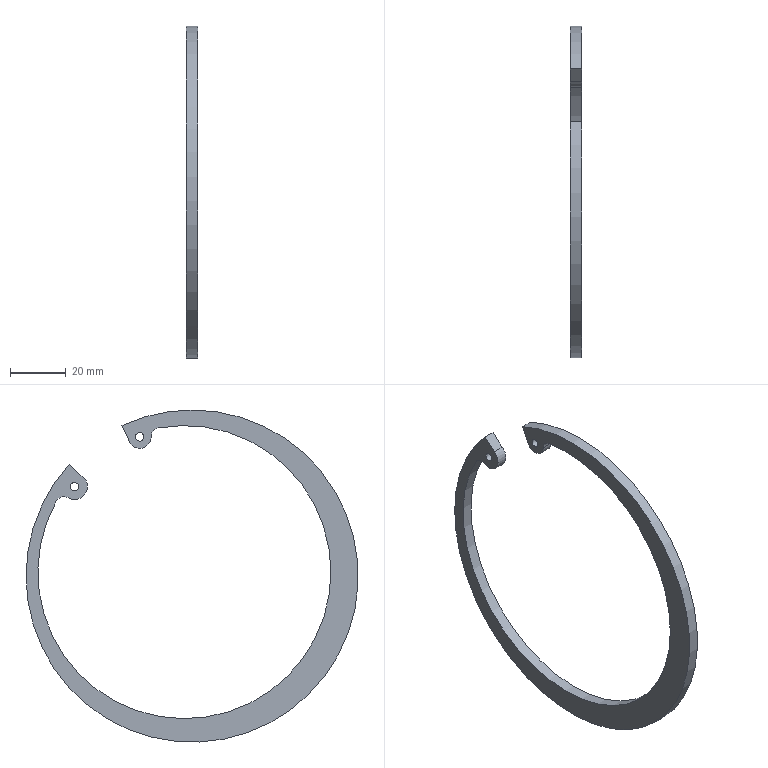Component | NX | HOLE_CLIP | 1 solid | 12 faces | box 4 x 119 x 119 mm | volume 9819 mm3 | cylinder 8 | plane 4 | commonest cylinder face diameters 6.15 x2 3 x2 8.2 x1 119 x1 9.272 x1 104.978 x1
STEP:
#1=CARTESIAN_POINT('',(0.,0.,0.));
#2=DIRECTION('',(0.,0.,1.));
#3=DIRECTION('',(1.,0.,0.));
#4=AXIS2_PLACEMENT_3D('',#1,#2,#3);
#5=CARTESIAN_POINT('',(1318.754,237.03,528.445));
#6=VERTEX_POINT('',#5);
#7=CARTESIAN_POINT('',(1314.754,237.03,528.445));
#8=VERTEX_POINT('',#7);
#9=CARTESIAN_POINT('',(1314.754,237.03,528.445));
#10=DIRECTION('',(-1.,0.,0.));
#11=VECTOR('',#10,1.);
#12=LINE('',#9,#11);
#13=CARTESIAN_POINT('',(1314.754,233.956,528.52));
#14=DIRECTION('',(1.,0.,0.));
#15=DIRECTION('',(0.,0.,-1.));
#16=AXIS2_PLACEMENT_3D('',#13,#14,#15);
#17=CYLINDRICAL_SURFACE('',#16,3.075);
#18=CARTESIAN_POINT('',(1.546,0.));
#19=DIRECTION('',(0.,-1.));
#20=VECTOR('',#19,1.);
#21=LINE('',#18,#20);
#22=(GEOMETRIC_REPRESENTATION_CONTEXT(2)PARAMETRIC_REPRESENTATION_CONTEXT()REPRESENTATION_CONTEXT('',''));
#23=DEFINITIONAL_REPRESENTATION('',(#21),#22);
#24=PCURVE('',#17,#23);
#25=CARTESIAN_POINT('',(1314.754,241.129,528.344));
#26=DIRECTION('',(1.,0.,0.));
#27=DIRECTION('',(0.,0.,-1.));
#28=AXIS2_PLACEMENT_3D('',#25,#26,#27);
#29=CYLINDRICAL_SURFACE('',#28,4.1);
#30=CARTESIAN_POINT('',(4.688,0.));
#31=DIRECTION('',(0.,-1.));
#32=VECTOR('',#31,1.);
#33=LINE('',#30,#32);
#34=(GEOMETRIC_REPRESENTATION_CONTEXT(2)PARAMETRIC_REPRESENTATION_CONTEXT()REPRESENTATION_CONTEXT('',''));
#35=DEFINITIONAL_REPRESENTATION('',(#33),#34);
#36=PCURVE('',#29,#35);
#37=SURFACE_CURVE('',#12,(#24,#36),.PCURVE_S1.);
#38=EDGE_CURVE('',#6,#8,#37,.T.);
#39=ORIENTED_EDGE('',*,*,#38,.T.);
#40=CARTESIAN_POINT('',(1314.754,234.507,531.545));
#41=VERTEX_POINT('',#40);
#42=CARTESIAN_POINT('',(1314.754,233.956,528.52));
#43=DIRECTION('',(1.,0.,0.));
#44=DIRECTION('',(0.,1.,0.));
#45=AXIS2_PLACEMENT_3D('',#42,#43,#44);
#46=CIRCLE('',#45,3.075);
#47=CARTESIAN_POINT('',(-4.712,0.));
#48=DIRECTION('',(1.,0.));
#49=VECTOR('',#48,1.);
#50=LINE('',#47,#49);
#51=(GEOMETRIC_REPRESENTATION_CONTEXT(2)PARAMETRIC_REPRESENTATION_CONTEXT()REPRESENTATION_CONTEXT('',''));
#52=DEFINITIONAL_REPRESENTATION('',(#50),#51);
#53=PCURVE('',#17,#52);
#54=CARTESIAN_POINT('',(1314.754,233.956,528.52));
#55=DIRECTION('',(-1.,0.,0.));
#56=DIRECTION('',(0.,0.,1.));
#57=AXIS2_PLACEMENT_3D('',#54,#55,#56);
#58=PLANE('',#57);
#59=CARTESIAN_POINT('',(0.,3.075));
#60=CARTESIAN_POINT('',(5.326,3.075));
#61=CARTESIAN_POINT('',(2.663,-1.538));
#62=CARTESIAN_POINT('',(0.,-6.15));
#63=CARTESIAN_POINT('',(-2.663,-1.538));
#64=CARTESIAN_POINT('',(-5.326,3.075));
#65=CARTESIAN_POINT('',(0.,3.075));
#66=(BOUNDED_CURVE()B_SPLINE_CURVE(2,(#59,#60,#61,#62,#63,#64,#65),.UNSPECIFIED.,.T.,.F.)B_SPLINE_CURVE_WITH_KNOTS((1,2,2,2,2,1),(-2.094,0.,2.094,4.189,6.283,8.378),.UNSPECIFIED.)CURVE()GEOMETRIC_REPRESENTATION_ITEM()RATIONAL_B_SPLINE_CURVE((1.,0.5,1.,0.5,1.,0.5,1.))REPRESENTATION_ITEM(''));
#67=(GEOMETRIC_REPRESENTATION_CONTEXT(2)PARAMETRIC_REPRESENTATION_CONTEXT()REPRESENTATION_CONTEXT('',''));
#68=DEFINITIONAL_REPRESENTATION('',(#66),#67);
#69=PCURVE('',#58,#68);
#70=SURFACE_CURVE('',#46,(#53,#69),.PCURVE_S1.);
#71=EDGE_CURVE('',#8,#41,#70,.T.);
#72=ORIENTED_EDGE('',*,*,#71,.T.);
#73=CARTESIAN_POINT('',(1318.754,234.507,531.545));
#74=VERTEX_POINT('',#73);
#75=CARTESIAN_POINT('',(1314.754,234.507,531.545));
#76=DIRECTION('',(-1.,0.,0.));
#77=VECTOR('',#76,1.);
#78=LINE('',#75,#77);
#79=CARTESIAN_POINT('',(2.962,0.));
#80=DIRECTION('',(0.,-1.));
#81=VECTOR('',#80,1.);
#82=LINE('',#79,#81);
#83=(GEOMETRIC_REPRESENTATION_CONTEXT(2)PARAMETRIC_REPRESENTATION_CONTEXT()REPRESENTATION_CONTEXT('',''));
#84=DEFINITIONAL_REPRESENTATION('',(#82),#83);
#85=PCURVE('',#17,#84);
#86=CARTESIAN_POINT('',(1314.754,225.111,479.904));
#87=DIRECTION('',(1.,0.,0.));
#88=DIRECTION('',(0.,0.,-1.));
#89=AXIS2_PLACEMENT_3D('',#86,#87,#88);
#90=CYLINDRICAL_SURFACE('',#89,52.489);
#91=CARTESIAN_POINT('',(2.962,0.));
#92=DIRECTION('',(0.,-1.));
#93=VECTOR('',#92,1.);
#94=LINE('',#91,#93);
#95=(GEOMETRIC_REPRESENTATION_CONTEXT(2)PARAMETRIC_REPRESENTATION_CONTEXT()REPRESENTATION_CONTEXT('',''));
#96=DEFINITIONAL_REPRESENTATION('',(#94),#95);
#97=PCURVE('',#90,#96);
#98=SURFACE_CURVE('',#78,(#85,#97),.PCURVE_S1.);
#99=EDGE_CURVE('',#74,#41,#98,.T.);
#100=ORIENTED_EDGE('',*,*,#99,.F.);
#101=CARTESIAN_POINT('',(1318.754,233.956,528.52));
#102=DIRECTION('',(1.,0.,0.));
#103=DIRECTION('',(0.,1.,0.));
#104=AXIS2_PLACEMENT_3D('',#101,#102,#103);
#105=CIRCLE('',#104,3.075);
#106=CARTESIAN_POINT('',(-4.712,4.));
#107=DIRECTION('',(1.,0.));
#108=VECTOR('',#107,1.);
#109=LINE('',#106,#108);
#110=(GEOMETRIC_REPRESENTATION_CONTEXT(2)PARAMETRIC_REPRESENTATION_CONTEXT()REPRESENTATION_CONTEXT('',''));
#111=DEFINITIONAL_REPRESENTATION('',(#109),#110);
#112=PCURVE('',#17,#111);
#113=CARTESIAN_POINT('',(1318.754,233.956,528.52));
#114=DIRECTION('',(-1.,0.,0.));
#115=DIRECTION('',(0.,0.,1.));
#116=AXIS2_PLACEMENT_3D('',#113,#114,#115);
#117=PLANE('',#116);
#118=CARTESIAN_POINT('',(0.,3.075));
#119=CARTESIAN_POINT('',(5.326,3.075));
#120=CARTESIAN_POINT('',(2.663,-1.538));
#121=CARTESIAN_POINT('',(0.,-6.15));
#122=CARTESIAN_POINT('',(-2.663,-1.538));
#123=CARTESIAN_POINT('',(-5.326,3.075));
#124=CARTESIAN_POINT('',(0.,3.075));
#125=(BOUNDED_CURVE()B_SPLINE_CURVE(2,(#118,#119,#120,#121,#122,#123,#124),.UNSPECIFIED.,.T.,.F.)B_SPLINE_CURVE_WITH_KNOTS((1,2,2,2,2,1),(-2.094,0.,2.094,4.189,6.283,8.378),.UNSPECIFIED.)CURVE()GEOMETRIC_REPRESENTATION_ITEM()RATIONAL_B_SPLINE_CURVE((1.,0.5,1.,0.5,1.,0.5,1.))REPRESENTATION_ITEM(''));
#126=(GEOMETRIC_REPRESENTATION_CONTEXT(2)PARAMETRIC_REPRESENTATION_CONTEXT()REPRESENTATION_CONTEXT('',''));
#127=DEFINITIONAL_REPRESENTATION('',(#125),#126);
#128=PCURVE('',#117,#127);
#129=SURFACE_CURVE('',#105,(#112,#128),.PCURVE_S1.);
#130=EDGE_CURVE('',#6,#74,#129,.T.);
#131=ORIENTED_EDGE('',*,*,#130,.F.);
#132=EDGE_LOOP('',(#39,#72,#100,#131));
#133=FACE_BOUND('',#132,.F.);
#134=ADVANCED_FACE('',(#133),#17,.F.);
#135=CARTESIAN_POINT('',(1318.754,244.461,525.955));
#136=VERTEX_POINT('',#135);
#137=CARTESIAN_POINT('',(1318.754,241.129,528.344));
#138=DIRECTION('',(-1.,0.,0.));
#139=DIRECTION('',(0.,1.,0.));
#140=AXIS2_PLACEMENT_3D('',#137,#138,#139);
#141=CIRCLE('',#140,4.1);
#142=CARTESIAN_POINT('',(7.854,4.));
#143=DIRECTION('',(-1.,0.));
#144=VECTOR('',#143,1.);
#145=LINE('',#142,#144);
#146=(GEOMETRIC_REPRESENTATION_CONTEXT(2)PARAMETRIC_REPRESENTATION_CONTEXT()REPRESENTATION_CONTEXT('',''));
#147=DEFINITIONAL_REPRESENTATION('',(#145),#146);
#148=PCURVE('',#29,#147);
#149=CARTESIAN_POINT('',(-0.1763,7.173));
#150=DIRECTION('',(0.,1.));
#151=AXIS2_PLACEMENT_2D('',#149,#150);
#152=CIRCLE('',#151,4.1);
#153=(GEOMETRIC_REPRESENTATION_CONTEXT(2)PARAMETRIC_REPRESENTATION_CONTEXT()REPRESENTATION_CONTEXT('',''));
#154=DEFINITIONAL_REPRESENTATION('',(#152),#153);
#155=PCURVE('',#117,#154);
#156=SURFACE_CURVE('',#141,(#148,#155),.PCURVE_S1.);
#157=EDGE_CURVE('',#136,#6,#156,.T.);
#158=ORIENTED_EDGE('',*,*,#157,.T.);
#159=ORIENTED_EDGE('',*,*,#38,.T.);
#160=CARTESIAN_POINT('',(1314.754,244.461,525.955));
#161=VERTEX_POINT('',#160);
#162=CARTESIAN_POINT('',(1314.754,241.129,528.344));
#163=DIRECTION('',(-1.,0.,0.));
#164=DIRECTION('',(0.,1.,0.));
#165=AXIS2_PLACEMENT_3D('',#162,#163,#164);
#166=CIRCLE('',#165,4.1);
#167=CARTESIAN_POINT('',(7.854,0.));
#168=DIRECTION('',(-1.,0.));
#169=VECTOR('',#168,1.);
#170=LINE('',#167,#169);
#171=(GEOMETRIC_REPRESENTATION_CONTEXT(2)PARAMETRIC_REPRESENTATION_CONTEXT()REPRESENTATION_CONTEXT('',''));
#172=DEFINITIONAL_REPRESENTATION('',(#170),#171);
#173=PCURVE('',#29,#172);
#174=CARTESIAN_POINT('',(-0.1763,7.173));
#175=DIRECTION('',(0.,1.));
#176=AXIS2_PLACEMENT_2D('',#174,#175);
#177=CIRCLE('',#176,4.1);
#178=(GEOMETRIC_REPRESENTATION_CONTEXT(2)PARAMETRIC_REPRESENTATION_CONTEXT()REPRESENTATION_CONTEXT('',''));
#179=DEFINITIONAL_REPRESENTATION('',(#177),#178);
#180=PCURVE('',#58,#179);
#181=SURFACE_CURVE('',#166,(#173,#180),.PCURVE_S1.);
#182=EDGE_CURVE('',#161,#8,#181,.T.);
#183=ORIENTED_EDGE('',*,*,#182,.F.);
#184=CARTESIAN_POINT('',(1314.754,244.461,525.955));
#185=DIRECTION('',(-1.,0.,0.));
#186=VECTOR('',#185,1.);
#187=LINE('',#184,#186);
#188=CARTESIAN_POINT('',(7.232,0.));
#189=DIRECTION('',(0.,-1.));
#190=VECTOR('',#189,1.);
#191=LINE('',#188,#190);
#192=(GEOMETRIC_REPRESENTATION_CONTEXT(2)PARAMETRIC_REPRESENTATION_CONTEXT()REPRESENTATION_CONTEXT('',''));
#193=DEFINITIONAL_REPRESENTATION('',(#191),#192);
#194=PCURVE('',#29,#193);
#195=CARTESIAN_POINT('',(1314.754,244.461,525.955));
#196=DIRECTION('',(0.,0.9065,-0.4222));
#197=DIRECTION('',(0.,0.4222,0.9065));
#198=AXIS2_PLACEMENT_3D('',#195,#196,#197);
#199=PLANE('',#198);
#200=CARTESIAN_POINT('',(0.,0.));
#201=DIRECTION('',(0.,-1.));
#202=VECTOR('',#201,1.);
#203=LINE('',#200,#202);
#204=(GEOMETRIC_REPRESENTATION_CONTEXT(2)PARAMETRIC_REPRESENTATION_CONTEXT()REPRESENTATION_CONTEXT('',''));
#205=DEFINITIONAL_REPRESENTATION('',(#203),#204);
#206=PCURVE('',#199,#205);
#207=SURFACE_CURVE('',#187,(#194,#206),.PCURVE_S1.);
#208=EDGE_CURVE('',#136,#161,#207,.T.);
#209=ORIENTED_EDGE('',*,*,#208,.F.);
#210=EDGE_LOOP('',(#158,#159,#183,#209));
#211=FACE_BOUND('',#210,.T.);
#212=ADVANCED_FACE('',(#211),#29,.T.);
#213=CARTESIAN_POINT('',(1318.754,247.47,532.414));
#214=VERTEX_POINT('',#213);
#215=CARTESIAN_POINT('',(1318.754,244.461,525.955));
#216=DIRECTION('',(0.,-0.4222,-0.9065));
#217=VECTOR('',#216,1.);
#218=LINE('',#215,#217);
#219=CARTESIAN_POINT('',(0.,4.));
#220=DIRECTION('',(-1.,0.));
#221=VECTOR('',#220,1.);
#222=LINE('',#219,#221);
#223=(GEOMETRIC_REPRESENTATION_CONTEXT(2)PARAMETRIC_REPRESENTATION_CONTEXT()REPRESENTATION_CONTEXT('',''));
#224=DEFINITIONAL_REPRESENTATION('',(#222),#223);
#225=PCURVE('',#199,#224);
#226=CARTESIAN_POINT('',(-2.565,10.505));
#227=DIRECTION('',(-0.9065,-0.4222));
#228=VECTOR('',#227,1.);
#229=LINE('',#226,#228);
#230=(GEOMETRIC_REPRESENTATION_CONTEXT(2)PARAMETRIC_REPRESENTATION_CONTEXT()REPRESENTATION_CONTEXT('',''));
#231=DEFINITIONAL_REPRESENTATION('',(#229),#230);
#232=PCURVE('',#117,#231);
#233=SURFACE_CURVE('',#218,(#225,#232),.PCURVE_S1.);
#234=EDGE_CURVE('',#214,#136,#233,.T.);
#235=ORIENTED_EDGE('',*,*,#234,.T.);
#236=ORIENTED_EDGE('',*,*,#208,.T.);
#237=CARTESIAN_POINT('',(1314.754,247.47,532.414));
#238=VERTEX_POINT('',#237);
#239=CARTESIAN_POINT('',(1314.754,244.461,525.955));
#240=DIRECTION('',(0.,-0.4222,-0.9065));
#241=VECTOR('',#240,1.);
#242=LINE('',#239,#241);
#243=CARTESIAN_POINT('',(0.,0.));
#244=DIRECTION('',(-1.,0.));
#245=VECTOR('',#244,1.);
#246=LINE('',#243,#245);
#247=(GEOMETRIC_REPRESENTATION_CONTEXT(2)PARAMETRIC_REPRESENTATION_CONTEXT()REPRESENTATION_CONTEXT('',''));
#248=DEFINITIONAL_REPRESENTATION('',(#246),#247);
#249=PCURVE('',#199,#248);
#250=CARTESIAN_POINT('',(-2.565,10.505));
#251=DIRECTION('',(-0.9065,-0.4222));
#252=VECTOR('',#251,1.);
#253=LINE('',#250,#252);
#254=(GEOMETRIC_REPRESENTATION_CONTEXT(2)PARAMETRIC_REPRESENTATION_CONTEXT()REPRESENTATION_CONTEXT('',''));
#255=DEFINITIONAL_REPRESENTATION('',(#253),#254);
#256=PCURVE('',#58,#255);
#257=SURFACE_CURVE('',#242,(#249,#256),.PCURVE_S1.);
#258=EDGE_CURVE('',#238,#161,#257,.T.);
#259=ORIENTED_EDGE('',*,*,#258,.F.);
#260=CARTESIAN_POINT('',(1314.754,247.47,532.414));
#261=DIRECTION('',(-1.,0.,0.));
#262=VECTOR('',#261,1.);
#263=LINE('',#260,#262);
#264=CARTESIAN_POINT('',(7.125,0.));
#265=DIRECTION('',(0.,-1.));
#266=VECTOR('',#265,1.);
#267=LINE('',#264,#266);
#268=(GEOMETRIC_REPRESENTATION_CONTEXT(2)PARAMETRIC_REPRESENTATION_CONTEXT()REPRESENTATION_CONTEXT('',''));
#269=DEFINITIONAL_REPRESENTATION('',(#267),#268);
#270=PCURVE('',#199,#269);
#271=CARTESIAN_POINT('',(1314.754,222.349,478.477));
#272=DIRECTION('',(1.,0.,0.));
#273=DIRECTION('',(0.,0.,-1.));
#274=AXIS2_PLACEMENT_3D('',#271,#272,#273);
#275=CYLINDRICAL_SURFACE('',#274,59.5);
#276=CARTESIAN_POINT('',(2.706,0.));
#277=DIRECTION('',(0.,-1.));
#278=VECTOR('',#277,1.);
#279=LINE('',#276,#278);
#280=(GEOMETRIC_REPRESENTATION_CONTEXT(2)PARAMETRIC_REPRESENTATION_CONTEXT()REPRESENTATION_CONTEXT('',''));
#281=DEFINITIONAL_REPRESENTATION('',(#279),#280);
#282=PCURVE('',#275,#281);
#283=SURFACE_CURVE('',#263,(#270,#282),.PCURVE_S1.);
#284=EDGE_CURVE('',#214,#238,#283,.T.);
#285=ORIENTED_EDGE('',*,*,#284,.F.);
#286=EDGE_LOOP('',(#235,#236,#259,#285));
#287=FACE_BOUND('',#286,.T.);
#288=ADVANCED_FACE('',(#287),#199,.T.);
#289=CARTESIAN_POINT('',(1318.754,266.41,518.464));
#290=VERTEX_POINT('',#289);
#291=CARTESIAN_POINT('',(1318.754,222.349,478.477));
#292=DIRECTION('',(-1.,0.,0.));
#293=DIRECTION('',(0.,1.,0.));
#294=AXIS2_PLACEMENT_3D('',#291,#292,#293);
#295=CIRCLE('',#294,59.5);
#296=CARTESIAN_POINT('',(14.137,4.));
#297=DIRECTION('',(-1.,0.));
#298=VECTOR('',#297,1.);
#299=LINE('',#296,#298);
#300=(GEOMETRIC_REPRESENTATION_CONTEXT(2)PARAMETRIC_REPRESENTATION_CONTEXT()REPRESENTATION_CONTEXT('',''));
#301=DEFINITIONAL_REPRESENTATION('',(#299),#300);
#302=PCURVE('',#275,#301);
#303=CARTESIAN_POINT('',(-50.043,-11.607));
#304=DIRECTION('',(0.,1.));
#305=AXIS2_PLACEMENT_2D('',#303,#304);
#306=CIRCLE('',#305,59.5);
#307=(GEOMETRIC_REPRESENTATION_CONTEXT(2)PARAMETRIC_REPRESENTATION_CONTEXT()REPRESENTATION_CONTEXT('',''));
#308=DEFINITIONAL_REPRESENTATION('',(#306),#307);
#309=PCURVE('',#117,#308);
#310=SURFACE_CURVE('',#295,(#302,#309),.PCURVE_S1.);
#311=EDGE_CURVE('',#290,#214,#310,.T.);
#312=ORIENTED_EDGE('',*,*,#311,.T.);
#313=ORIENTED_EDGE('',*,*,#284,.T.);
#314=CARTESIAN_POINT('',(1314.754,266.41,518.464));
#315=VERTEX_POINT('',#314);
#316=CARTESIAN_POINT('',(1314.754,222.349,478.477));
#317=DIRECTION('',(-1.,0.,0.));
#318=DIRECTION('',(0.,1.,0.));
#319=AXIS2_PLACEMENT_3D('',#316,#317,#318);
#320=CIRCLE('',#319,59.5);
#321=CARTESIAN_POINT('',(14.137,0.));
#322=DIRECTION('',(-1.,0.));
#323=VECTOR('',#322,1.);
#324=LINE('',#321,#323);
#325=(GEOMETRIC_REPRESENTATION_CONTEXT(2)PARAMETRIC_REPRESENTATION_CONTEXT()REPRESENTATION_CONTEXT('',''));
#326=DEFINITIONAL_REPRESENTATION('',(#324),#325);
#327=PCURVE('',#275,#326);
#328=CARTESIAN_POINT('',(-50.043,-11.607));
#329=DIRECTION('',(0.,1.));
#330=AXIS2_PLACEMENT_2D('',#328,#329);
#331=CIRCLE('',#330,59.5);
#332=(GEOMETRIC_REPRESENTATION_CONTEXT(2)PARAMETRIC_REPRESENTATION_CONTEXT()REPRESENTATION_CONTEXT('',''));
#333=DEFINITIONAL_REPRESENTATION('',(#331),#332);
#334=PCURVE('',#58,#333);
#335=SURFACE_CURVE('',#320,(#327,#334),.PCURVE_S1.);
#336=EDGE_CURVE('',#315,#238,#335,.T.);
#337=ORIENTED_EDGE('',*,*,#336,.F.);
#338=CARTESIAN_POINT('',(1314.754,266.41,518.464));
#339=DIRECTION('',(-1.,0.,0.));
#340=VECTOR('',#339,1.);
#341=LINE('',#338,#340);
#342=CARTESIAN_POINT('',(8.591,0.));
#343=DIRECTION('',(0.,-1.));
#344=VECTOR('',#343,1.);
#345=LINE('',#342,#344);
#346=(GEOMETRIC_REPRESENTATION_CONTEXT(2)PARAMETRIC_REPRESENTATION_CONTEXT()REPRESENTATION_CONTEXT('',''));
#347=DEFINITIONAL_REPRESENTATION('',(#345),#346);
#348=PCURVE('',#275,#347);
#349=CARTESIAN_POINT('',(1314.754,266.41,518.464));
#350=DIRECTION('',(0.,-0.672,0.7405));
#351=DIRECTION('',(0.,-0.7405,-0.672));
#352=AXIS2_PLACEMENT_3D('',#349,#350,#351);
#353=PLANE('',#352);
#354=CARTESIAN_POINT('',(0.,0.));
#355=DIRECTION('',(0.,-1.));
#356=VECTOR('',#355,1.);
#357=LINE('',#354,#356);
#358=(GEOMETRIC_REPRESENTATION_CONTEXT(2)PARAMETRIC_REPRESENTATION_CONTEXT()REPRESENTATION_CONTEXT('',''));
#359=DEFINITIONAL_REPRESENTATION('',(#357),#358);
#360=PCURVE('',#353,#359);
#361=SURFACE_CURVE('',#341,(#348,#360),.PCURVE_S1.);
#362=EDGE_CURVE('',#290,#315,#361,.T.);
#363=ORIENTED_EDGE('',*,*,#362,.F.);
#364=EDGE_LOOP('',(#312,#313,#337,#363));
#365=FACE_BOUND('',#364,.T.);
#366=ADVANCED_FACE('',(#365),#275,.T.);
#367=CARTESIAN_POINT('',(1318.754,261.776,514.258));
#368=VERTEX_POINT('',#367);
#369=CARTESIAN_POINT('',(1318.754,266.41,518.464));
#370=DIRECTION('',(-0.,0.7405,0.672));
#371=VECTOR('',#370,1.);
#372=LINE('',#369,#371);
#373=CARTESIAN_POINT('',(0.,4.));
#374=DIRECTION('',(-1.,-0.));
#375=VECTOR('',#374,1.);
#376=LINE('',#373,#375);
#377=(GEOMETRIC_REPRESENTATION_CONTEXT(2)PARAMETRIC_REPRESENTATION_CONTEXT()REPRESENTATION_CONTEXT('',''));
#378=DEFINITIONAL_REPRESENTATION('',(#376),#377);
#379=PCURVE('',#353,#378);
#380=CARTESIAN_POINT('',(-10.056,32.453));
#381=DIRECTION('',(0.672,0.7405));
#382=VECTOR('',#381,1.);
#383=LINE('',#380,#382);
#384=(GEOMETRIC_REPRESENTATION_CONTEXT(2)PARAMETRIC_REPRESENTATION_CONTEXT()REPRESENTATION_CONTEXT('',''));
#385=DEFINITIONAL_REPRESENTATION('',(#383),#384);
#386=PCURVE('',#117,#385);
#387=SURFACE_CURVE('',#372,(#379,#386),.PCURVE_S1.);
#388=EDGE_CURVE('',#368,#290,#387,.T.);
#389=ORIENTED_EDGE('',*,*,#388,.T.);
#390=ORIENTED_EDGE('',*,*,#362,.T.);
#391=CARTESIAN_POINT('',(1314.754,261.776,514.258));
#392=VERTEX_POINT('',#391);
#393=CARTESIAN_POINT('',(1314.754,266.41,518.464));
#394=DIRECTION('',(-0.,0.7405,0.672));
#395=VECTOR('',#394,1.);
#396=LINE('',#393,#395);
#397=CARTESIAN_POINT('',(0.,0.));
#398=DIRECTION('',(-1.,-0.));
#399=VECTOR('',#398,1.);
#400=LINE('',#397,#399);
#401=(GEOMETRIC_REPRESENTATION_CONTEXT(2)PARAMETRIC_REPRESENTATION_CONTEXT()REPRESENTATION_CONTEXT('',''));
#402=DEFINITIONAL_REPRESENTATION('',(#400),#401);
#403=PCURVE('',#353,#402);
#404=CARTESIAN_POINT('',(-10.056,32.453));
#405=DIRECTION('',(0.672,0.7405));
#406=VECTOR('',#405,1.);
#407=LINE('',#404,#406);
#408=(GEOMETRIC_REPRESENTATION_CONTEXT(2)PARAMETRIC_REPRESENTATION_CONTEXT()REPRESENTATION_CONTEXT('',''));
#409=DEFINITIONAL_REPRESENTATION('',(#407),#408);
#410=PCURVE('',#58,#409);
#411=SURFACE_CURVE('',#396,(#403,#410),.PCURVE_S1.);
#412=EDGE_CURVE('',#392,#315,#411,.T.);
#413=ORIENTED_EDGE('',*,*,#412,.F.);
#414=CARTESIAN_POINT('',(1314.754,261.776,514.258));
#415=DIRECTION('',(-1.,0.,0.));
#416=VECTOR('',#415,1.);
#417=LINE('',#414,#416);
#418=CARTESIAN_POINT('',(6.258,0.));
#419=DIRECTION('',(0.,-1.));
#420=VECTOR('',#419,1.);
#421=LINE('',#418,#420);
#422=(GEOMETRIC_REPRESENTATION_CONTEXT(2)PARAMETRIC_REPRESENTATION_CONTEXT()REPRESENTATION_CONTEXT('',''));
#423=DEFINITIONAL_REPRESENTATION('',(#421),#422);
#424=PCURVE('',#353,#423);
#425=CARTESIAN_POINT('',(1314.754,264.515,510.518));
#426=DIRECTION('',(1.,0.,0.));
#427=DIRECTION('',(0.,0.,-1.));
#428=AXIS2_PLACEMENT_3D('',#425,#426,#427);
#429=CYLINDRICAL_SURFACE('',#428,4.636);
#430=CARTESIAN_POINT('',(3.774,0.));
#431=DIRECTION('',(0.,-1.));
#432=VECTOR('',#431,1.);
#433=LINE('',#430,#432);
#434=(GEOMETRIC_REPRESENTATION_CONTEXT(2)PARAMETRIC_REPRESENTATION_CONTEXT()REPRESENTATION_CONTEXT('',''));
#435=DEFINITIONAL_REPRESENTATION('',(#433),#434);
#436=PCURVE('',#429,#435);
#437=SURFACE_CURVE('',#417,(#424,#436),.PCURVE_S1.);
#438=EDGE_CURVE('',#368,#392,#437,.T.);
#439=ORIENTED_EDGE('',*,*,#438,.F.);
#440=EDGE_LOOP('',(#389,#390,#413,#439));
#441=FACE_BOUND('',#440,.T.);
#442=ADVANCED_FACE('',(#441),#353,.T.);
#443=CARTESIAN_POINT('',(1318.754,267.254,506.778));
#444=VERTEX_POINT('',#443);
#445=CARTESIAN_POINT('',(1318.754,264.515,510.518));
#446=DIRECTION('',(-1.,0.,0.));
#447=DIRECTION('',(0.,1.,0.));
#448=AXIS2_PLACEMENT_3D('',#445,#446,#447);
#449=CIRCLE('',#448,4.636);
#450=CARTESIAN_POINT('',(7.854,4.));
#451=DIRECTION('',(-1.,0.));
#452=VECTOR('',#451,1.);
#453=LINE('',#450,#452);
#454=(GEOMETRIC_REPRESENTATION_CONTEXT(2)PARAMETRIC_REPRESENTATION_CONTEXT()REPRESENTATION_CONTEXT('',''));
#455=DEFINITIONAL_REPRESENTATION('',(#453),#454);
#456=PCURVE('',#429,#455);
#457=CARTESIAN_POINT('',(-18.002,30.559));
#458=DIRECTION('',(0.,1.));
#459=AXIS2_PLACEMENT_2D('',#457,#458);
#460=CIRCLE('',#459,4.636);
#461=(GEOMETRIC_REPRESENTATION_CONTEXT(2)PARAMETRIC_REPRESENTATION_CONTEXT()REPRESENTATION_CONTEXT('',''));
#462=DEFINITIONAL_REPRESENTATION('',(#460),#461);
#463=PCURVE('',#117,#462);
#464=SURFACE_CURVE('',#449,(#456,#463),.PCURVE_S1.);
#465=EDGE_CURVE('',#444,#368,#464,.T.);
#466=ORIENTED_EDGE('',*,*,#465,.T.);
#467=ORIENTED_EDGE('',*,*,#438,.T.);
#468=CARTESIAN_POINT('',(1314.754,267.254,506.778));
#469=VERTEX_POINT('',#468);
#470=CARTESIAN_POINT('',(1314.754,264.515,510.518));
#471=DIRECTION('',(-1.,0.,0.));
#472=DIRECTION('',(0.,1.,0.));
#473=AXIS2_PLACEMENT_3D('',#470,#471,#472);
#474=CIRCLE('',#473,4.636);
#475=CARTESIAN_POINT('',(7.854,0.));
#476=DIRECTION('',(-1.,0.));
#477=VECTOR('',#476,1.);
#478=LINE('',#475,#477);
#479=(GEOMETRIC_REPRESENTATION_CONTEXT(2)PARAMETRIC_REPRESENTATION_CONTEXT()REPRESENTATION_CONTEXT('',''));
#480=DEFINITIONAL_REPRESENTATION('',(#478),#479);
#481=PCURVE('',#429,#480);
#482=CARTESIAN_POINT('',(-18.002,30.559));
#483=DIRECTION('',(0.,1.));
#484=AXIS2_PLACEMENT_2D('',#482,#483);
#485=CIRCLE('',#484,4.636);
#486=(GEOMETRIC_REPRESENTATION_CONTEXT(2)PARAMETRIC_REPRESENTATION_CONTEXT()REPRESENTATION_CONTEXT('',''));
#487=DEFINITIONAL_REPRESENTATION('',(#485),#486);
#488=PCURVE('',#58,#487);
#489=SURFACE_CURVE('',#474,(#481,#488),.PCURVE_S1.);
#490=EDGE_CURVE('',#469,#392,#489,.T.);
#491=ORIENTED_EDGE('',*,*,#490,.F.);
#492=CARTESIAN_POINT('',(1314.754,267.254,506.778));
#493=DIRECTION('',(-1.,0.,0.));
#494=VECTOR('',#493,1.);
#495=LINE('',#492,#494);
#496=CARTESIAN_POINT('',(6.915,0.));
#497=DIRECTION('',(0.,-1.));
#498=VECTOR('',#497,1.);
#499=LINE('',#496,#498);
#500=(GEOMETRIC_REPRESENTATION_CONTEXT(2)PARAMETRIC_REPRESENTATION_CONTEXT()REPRESENTATION_CONTEXT('',''));
#501=DEFINITIONAL_REPRESENTATION('',(#499),#500);
#502=PCURVE('',#429,#501);
#503=CARTESIAN_POINT('',(1314.754,268.313,503.891));
#504=DIRECTION('',(1.,0.,0.));
#505=DIRECTION('',(0.,0.,-1.));
#506=AXIS2_PLACEMENT_3D('',#503,#504,#505);
#507=CYLINDRICAL_SURFACE('',#506,3.075);
#508=CARTESIAN_POINT('',(3.493,0.));
#509=DIRECTION('',(0.,-1.));
#510=VECTOR('',#509,1.);
#511=LINE('',#508,#510);
#512=(GEOMETRIC_REPRESENTATION_CONTEXT(2)PARAMETRIC_REPRESENTATION_CONTEXT()REPRESENTATION_CONTEXT('',''));
#513=DEFINITIONAL_REPRESENTATION('',(#511),#512);
#514=PCURVE('',#507,#513);
#515=SURFACE_CURVE('',#495,(#502,#514),.PCURVE_S1.);
#516=EDGE_CURVE('',#444,#469,#515,.T.);
#517=ORIENTED_EDGE('',*,*,#516,.F.);
#518=EDGE_LOOP('',(#466,#467,#491,#517));
#519=FACE_BOUND('',#518,.T.);
#520=ADVANCED_FACE('',(#519),#429,.T.);
#521=CARTESIAN_POINT('',(1318.754,271.001,505.383));
#522=VERTEX_POINT('',#521);
#523=CARTESIAN_POINT('',(1314.754,271.001,505.383));
#524=VERTEX_POINT('',#523);
#525=CARTESIAN_POINT('',(1314.754,271.001,505.383));
#526=DIRECTION('',(-1.,0.,0.));
#527=VECTOR('',#526,1.);
#528=LINE('',#525,#527);
#529=CARTESIAN_POINT('',(2.078,0.));
#530=DIRECTION('',(0.,-1.));
#531=VECTOR('',#530,1.);
#532=LINE('',#529,#531);
#533=(GEOMETRIC_REPRESENTATION_CONTEXT(2)PARAMETRIC_REPRESENTATION_CONTEXT()REPRESENTATION_CONTEXT('',''));
#534=DEFINITIONAL_REPRESENTATION('',(#532),#533);
#535=PCURVE('',#507,#534);
#536=CARTESIAN_POINT('',(8.361,0.));
#537=DIRECTION('',(0.,-1.));
#538=VECTOR('',#537,1.);
#539=LINE('',#536,#538);
#540=(GEOMETRIC_REPRESENTATION_CONTEXT(2)PARAMETRIC_REPRESENTATION_CONTEXT()REPRESENTATION_CONTEXT('',''));
#541=DEFINITIONAL_REPRESENTATION('',(#539),#540);
#542=PCURVE('',#90,#541);
#543=SURFACE_CURVE('',#528,(#535,#542),.PCURVE_S1.);
#544=EDGE_CURVE('',#522,#524,#543,.T.);
#545=ORIENTED_EDGE('',*,*,#544,.T.);
#546=CARTESIAN_POINT('',(1314.754,268.313,503.891));
#547=DIRECTION('',(1.,0.,0.));
#548=DIRECTION('',(0.,1.,0.));
#549=AXIS2_PLACEMENT_3D('',#546,#547,#548);
#550=CIRCLE('',#549,3.075);
#551=CARTESIAN_POINT('',(1.571,0.));
#552=DIRECTION('',(1.,0.));
#553=VECTOR('',#552,1.);
#554=LINE('',#551,#553);
#555=(GEOMETRIC_REPRESENTATION_CONTEXT(2)PARAMETRIC_REPRESENTATION_CONTEXT()REPRESENTATION_CONTEXT('',''));
#556=DEFINITIONAL_REPRESENTATION('',(#554),#555);
#557=PCURVE('',#507,#556);
#558=CARTESIAN_POINT('',(-24.63,37.432));
#559=CARTESIAN_POINT('',(-19.303,37.432));
#560=CARTESIAN_POINT('',(-21.966,32.819));
#561=CARTESIAN_POINT('',(-24.63,28.207));
#562=CARTESIAN_POINT('',(-27.293,32.819));
#563=CARTESIAN_POINT('',(-29.956,37.432));
#564=CARTESIAN_POINT('',(-24.63,37.432));
#565=(BOUNDED_CURVE()B_SPLINE_CURVE(2,(#558,#559,#560,#561,#562,#563,#564),.UNSPECIFIED.,.T.,.F.)B_SPLINE_CURVE_WITH_KNOTS((1,2,2,2,2,1),(-2.094,0.,2.094,4.189,6.283,8.378),.UNSPECIFIED.)CURVE()GEOMETRIC_REPRESENTATION_ITEM()RATIONAL_B_SPLINE_CURVE((1.,0.5,1.,0.5,1.,0.5,1.))REPRESENTATION_ITEM(''));
#566=(GEOMETRIC_REPRESENTATION_CONTEXT(2)PARAMETRIC_REPRESENTATION_CONTEXT()REPRESENTATION_CONTEXT('',''));
#567=DEFINITIONAL_REPRESENTATION('',(#565),#566);
#568=PCURVE('',#58,#567);
#569=SURFACE_CURVE('',#550,(#557,#568),.PCURVE_S1.);
#570=EDGE_CURVE('',#524,#469,#569,.T.);
#571=ORIENTED_EDGE('',*,*,#570,.T.);
#572=ORIENTED_EDGE('',*,*,#516,.F.);
#573=CARTESIAN_POINT('',(1318.754,268.313,503.891));
#574=DIRECTION('',(1.,0.,0.));
#575=DIRECTION('',(0.,1.,0.));
#576=AXIS2_PLACEMENT_3D('',#573,#574,#575);
#577=CIRCLE('',#576,3.075);
#578=CARTESIAN_POINT('',(1.571,4.));
#579=DIRECTION('',(1.,0.));
#580=VECTOR('',#579,1.);
#581=LINE('',#578,#580);
#582=(GEOMETRIC_REPRESENTATION_CONTEXT(2)PARAMETRIC_REPRESENTATION_CONTEXT()REPRESENTATION_CONTEXT('',''));
#583=DEFINITIONAL_REPRESENTATION('',(#581),#582);
#584=PCURVE('',#507,#583);
#585=CARTESIAN_POINT('',(-24.63,37.432));
#586=CARTESIAN_POINT('',(-19.303,37.432));
#587=CARTESIAN_POINT('',(-21.966,32.819));
#588=CARTESIAN_POINT('',(-24.63,28.207));
#589=CARTESIAN_POINT('',(-27.293,32.819));
#590=CARTESIAN_POINT('',(-29.956,37.432));
#591=CARTESIAN_POINT('',(-24.63,37.432));
#592=(BOUNDED_CURVE()B_SPLINE_CURVE(2,(#585,#586,#587,#588,#589,#590,#591),.UNSPECIFIED.,.T.,.F.)B_SPLINE_CURVE_WITH_KNOTS((1,2,2,2,2,1),(-2.094,0.,2.094,4.189,6.283,8.378),.UNSPECIFIED.)CURVE()GEOMETRIC_REPRESENTATION_ITEM()RATIONAL_B_SPLINE_CURVE((1.,0.5,1.,0.5,1.,0.5,1.))REPRESENTATION_ITEM(''));
#593=(GEOMETRIC_REPRESENTATION_CONTEXT(2)PARAMETRIC_REPRESENTATION_CONTEXT()REPRESENTATION_CONTEXT('',''));
#594=DEFINITIONAL_REPRESENTATION('',(#592),#593);
#595=PCURVE('',#117,#594);
#596=SURFACE_CURVE('',#577,(#584,#595),.PCURVE_S1.);
#597=EDGE_CURVE('',#522,#444,#596,.T.);
#598=ORIENTED_EDGE('',*,*,#597,.F.);
#599=EDGE_LOOP('',(#545,#571,#572,#598));
#600=FACE_BOUND('',#599,.F.);
#601=ADVANCED_FACE('',(#600),#507,.F.);
#602=CARTESIAN_POINT('',(1314.754,242.629,528.344));
#603=VERTEX_POINT('',#602);
#604=CARTESIAN_POINT('',(1314.754,241.129,528.344));
#605=DIRECTION('',(-1.,0.,0.));
#606=DIRECTION('',(0.,1.,0.));
#607=AXIS2_PLACEMENT_3D('',#604,#605,#606);
#608=CIRCLE('',#607,1.5);
#609=CARTESIAN_POINT('',(1314.754,241.129,528.344));
#610=DIRECTION('',(1.,0.,0.));
#611=DIRECTION('',(0.,0.,-1.));
#612=AXIS2_PLACEMENT_3D('',#609,#610,#611);
#613=CYLINDRICAL_SURFACE('',#612,1.5);
#614=CARTESIAN_POINT('',(7.854,0.));
#615=DIRECTION('',(-1.,0.));
#616=VECTOR('',#615,1.);
#617=LINE('',#614,#616);
#618=(GEOMETRIC_REPRESENTATION_CONTEXT(2)PARAMETRIC_REPRESENTATION_CONTEXT()REPRESENTATION_CONTEXT('',''));
#619=DEFINITIONAL_REPRESENTATION('',(#617),#618);
#620=PCURVE('',#613,#619);
#621=CARTESIAN_POINT('',(-0.1763,7.173));
#622=DIRECTION('',(0.,1.));
#623=AXIS2_PLACEMENT_2D('',#621,#622);
#624=CIRCLE('',#623,1.5);
#625=(GEOMETRIC_REPRESENTATION_CONTEXT(2)PARAMETRIC_REPRESENTATION_CONTEXT()REPRESENTATION_CONTEXT('',''));
#626=DEFINITIONAL_REPRESENTATION('',(#624),#625);
#627=PCURVE('',#58,#626);
#628=SURFACE_CURVE('',#608,(#620,#627),.PCURVE_S1.);
#629=EDGE_CURVE('',#603,#603,#628,.T.);
#630=ORIENTED_EDGE('',*,*,#629,.F.);
#631=CARTESIAN_POINT('',(1318.754,242.629,528.344));
#632=VERTEX_POINT('',#631);
#633=CARTESIAN_POINT('',(1314.754,242.629,528.344));
#634=CARTESIAN_POINT('',(1318.754,242.629,528.344));
#635=B_SPLINE_CURVE_WITH_KNOTS('',1,(#633,#634),.UNSPECIFIED.,.F.,.F.,(2,2),(0.,4.),.PIECEWISE_BEZIER_KNOTS.);
#636=CARTESIAN_POINT('',(7.854,0.));
#637=DIRECTION('',(0.,1.));
#638=VECTOR('',#637,1.);
#639=LINE('',#636,#638);
#640=(GEOMETRIC_REPRESENTATION_CONTEXT(2)PARAMETRIC_REPRESENTATION_CONTEXT()REPRESENTATION_CONTEXT('',''));
#641=DEFINITIONAL_REPRESENTATION('',(#639),#640);
#642=PCURVE('',#613,#641);
#643=CARTESIAN_POINT('',(1.571,0.));
#644=DIRECTION('',(0.,1.));
#645=VECTOR('',#644,1.);
#646=LINE('',#643,#645);
#647=(GEOMETRIC_REPRESENTATION_CONTEXT(2)PARAMETRIC_REPRESENTATION_CONTEXT()REPRESENTATION_CONTEXT('',''));
#648=DEFINITIONAL_REPRESENTATION('',(#646),#647);
#649=PCURVE('',#613,#648);
#650=SEAM_CURVE('',#635,(#642,#649),.PCURVE_S1.);
#651=EDGE_CURVE('',#603,#632,#650,.T.);
#652=ORIENTED_EDGE('',*,*,#651,.T.);
#653=CARTESIAN_POINT('',(1318.754,241.129,528.344));
#654=DIRECTION('',(-1.,0.,0.));
#655=DIRECTION('',(0.,1.,0.));
#656=AXIS2_PLACEMENT_3D('',#653,#654,#655);
#657=CIRCLE('',#656,1.5);
#658=CARTESIAN_POINT('',(7.854,4.));
#659=DIRECTION('',(-1.,0.));
#660=VECTOR('',#659,1.);
#661=LINE('',#658,#660);
#662=(GEOMETRIC_REPRESENTATION_CONTEXT(2)PARAMETRIC_REPRESENTATION_CONTEXT()REPRESENTATION_CONTEXT('',''));
#663=DEFINITIONAL_REPRESENTATION('',(#661),#662);
#664=PCURVE('',#613,#663);
#665=CARTESIAN_POINT('',(-0.1763,7.173));
#666=DIRECTION('',(0.,1.));
#667=AXIS2_PLACEMENT_2D('',#665,#666);
#668=CIRCLE('',#667,1.5);
#669=(GEOMETRIC_REPRESENTATION_CONTEXT(2)PARAMETRIC_REPRESENTATION_CONTEXT()REPRESENTATION_CONTEXT('',''));
#670=DEFINITIONAL_REPRESENTATION('',(#668),#669);
#671=PCURVE('',#117,#670);
#672=SURFACE_CURVE('',#657,(#664,#671),.PCURVE_S1.);
#673=EDGE_CURVE('',#632,#632,#672,.T.);
#674=ORIENTED_EDGE('',*,*,#673,.T.);
#675=ORIENTED_EDGE('',*,*,#651,.F.);
#676=EDGE_LOOP('',(#630,#652,#674,#675));
#677=FACE_BOUND('',#676,.F.);
#678=ADVANCED_FACE('',(#677),#613,.F.);
#679=ORIENTED_EDGE('',*,*,#99,.T.);
#680=CARTESIAN_POINT('',(1314.754,225.111,479.904));
#681=DIRECTION('',(1.,0.,0.));
#682=DIRECTION('',(0.,1.,0.));
#683=AXIS2_PLACEMENT_3D('',#680,#681,#682);
#684=CIRCLE('',#683,52.489);
#685=CARTESIAN_POINT('',(1.571,0.));
#686=DIRECTION('',(1.,0.));
#687=VECTOR('',#686,1.);
#688=LINE('',#685,#687);
#689=(GEOMETRIC_REPRESENTATION_CONTEXT(2)PARAMETRIC_REPRESENTATION_CONTEXT()REPRESENTATION_CONTEXT('',''));
#690=DEFINITIONAL_REPRESENTATION('',(#688),#689);
#691=PCURVE('',#90,#690);
#692=CARTESIAN_POINT('',(-48.616,43.644));
#693=CARTESIAN_POINT('',(42.298,43.644));
#694=CARTESIAN_POINT('',(-3.159,-35.09));
#695=CARTESIAN_POINT('',(-48.616,-113.823));
#696=CARTESIAN_POINT('',(-94.072,-35.09));
#697=CARTESIAN_POINT('',(-139.529,43.644));
#698=CARTESIAN_POINT('',(-48.616,43.644));
#699=(BOUNDED_CURVE()B_SPLINE_CURVE(2,(#692,#693,#694,#695,#696,#697,#698),.UNSPECIFIED.,.T.,.F.)B_SPLINE_CURVE_WITH_KNOTS((1,2,2,2,2,1),(-2.094,0.,2.094,4.189,6.283,8.378),.UNSPECIFIED.)CURVE()GEOMETRIC_REPRESENTATION_ITEM()RATIONAL_B_SPLINE_CURVE((1.,0.5,1.,0.5,1.,0.5,1.))REPRESENTATION_ITEM(''));
#700=(GEOMETRIC_REPRESENTATION_CONTEXT(2)PARAMETRIC_REPRESENTATION_CONTEXT()REPRESENTATION_CONTEXT('',''));
#701=DEFINITIONAL_REPRESENTATION('',(#699),#700);
#702=PCURVE('',#58,#701);
#703=SURFACE_CURVE('',#684,(#691,#702),.PCURVE_S1.);
#704=EDGE_CURVE('',#41,#524,#703,.T.);
#705=ORIENTED_EDGE('',*,*,#704,.T.);
#706=ORIENTED_EDGE('',*,*,#544,.F.);
#707=CARTESIAN_POINT('',(1318.754,225.111,479.904));
#708=DIRECTION('',(1.,0.,0.));
#709=DIRECTION('',(0.,1.,0.));
#710=AXIS2_PLACEMENT_3D('',#707,#708,#709);
#711=CIRCLE('',#710,52.489);
#712=CARTESIAN_POINT('',(1.571,4.));
#713=DIRECTION('',(1.,0.));
#714=VECTOR('',#713,1.);
#715=LINE('',#712,#714);
#716=(GEOMETRIC_REPRESENTATION_CONTEXT(2)PARAMETRIC_REPRESENTATION_CONTEXT()REPRESENTATION_CONTEXT('',''));
#717=DEFINITIONAL_REPRESENTATION('',(#715),#716);
#718=PCURVE('',#90,#717);
#719=CARTESIAN_POINT('',(-48.616,43.644));
#720=CARTESIAN_POINT('',(42.298,43.644));
#721=CARTESIAN_POINT('',(-3.159,-35.09));
#722=CARTESIAN_POINT('',(-48.616,-113.823));
#723=CARTESIAN_POINT('',(-94.072,-35.09));
#724=CARTESIAN_POINT('',(-139.529,43.644));
#725=CARTESIAN_POINT('',(-48.616,43.644));
#726=(BOUNDED_CURVE()B_SPLINE_CURVE(2,(#719,#720,#721,#722,#723,#724,#725),.UNSPECIFIED.,.T.,.F.)B_SPLINE_CURVE_WITH_KNOTS((1,2,2,2,2,1),(-2.094,0.,2.094,4.189,6.283,8.378),.UNSPECIFIED.)CURVE()GEOMETRIC_REPRESENTATION_ITEM()RATIONAL_B_SPLINE_CURVE((1.,0.5,1.,0.5,1.,0.5,1.))REPRESENTATION_ITEM(''));
#727=(GEOMETRIC_REPRESENTATION_CONTEXT(2)PARAMETRIC_REPRESENTATION_CONTEXT()REPRESENTATION_CONTEXT('',''));
#728=DEFINITIONAL_REPRESENTATION('',(#726),#727);
#729=PCURVE('',#117,#728);
#730=SURFACE_CURVE('',#711,(#718,#729),.PCURVE_S1.);
#731=EDGE_CURVE('',#74,#522,#730,.T.);
#732=ORIENTED_EDGE('',*,*,#731,.F.);
#733=EDGE_LOOP('',(#679,#705,#706,#732));
#734=FACE_BOUND('',#733,.F.);
#735=ADVANCED_FACE('',(#734),#90,.F.);
#736=CARTESIAN_POINT('',(1314.754,266.015,510.518));
#737=VERTEX_POINT('',#736);
#738=CARTESIAN_POINT('',(1314.754,264.515,510.518));
#739=DIRECTION('',(-1.,0.,0.));
#740=DIRECTION('',(0.,1.,0.));
#741=AXIS2_PLACEMENT_3D('',#738,#739,#740);
#742=CIRCLE('',#741,1.5);
#743=CARTESIAN_POINT('',(1314.754,264.515,510.518));
#744=DIRECTION('',(1.,0.,0.));
#745=DIRECTION('',(0.,0.,-1.));
#746=AXIS2_PLACEMENT_3D('',#743,#744,#745);
#747=CYLINDRICAL_SURFACE('',#746,1.5);
#748=CARTESIAN_POINT('',(7.854,0.));
#749=DIRECTION('',(-1.,0.));
#750=VECTOR('',#749,1.);
#751=LINE('',#748,#750);
#752=(GEOMETRIC_REPRESENTATION_CONTEXT(2)PARAMETRIC_REPRESENTATION_CONTEXT()REPRESENTATION_CONTEXT('',''));
#753=DEFINITIONAL_REPRESENTATION('',(#751),#752);
#754=PCURVE('',#747,#753);
#755=CARTESIAN_POINT('',(-18.002,30.559));
#756=DIRECTION('',(0.,1.));
#757=AXIS2_PLACEMENT_2D('',#755,#756);
#758=CIRCLE('',#757,1.5);
#759=(GEOMETRIC_REPRESENTATION_CONTEXT(2)PARAMETRIC_REPRESENTATION_CONTEXT()REPRESENTATION_CONTEXT('',''));
#760=DEFINITIONAL_REPRESENTATION('',(#758),#759);
#761=PCURVE('',#58,#760);
#762=SURFACE_CURVE('',#742,(#754,#761),.PCURVE_S1.);
#763=EDGE_CURVE('',#737,#737,#762,.T.);
#764=ORIENTED_EDGE('',*,*,#763,.F.);
#765=CARTESIAN_POINT('',(1318.754,266.015,510.518));
#766=VERTEX_POINT('',#765);
#767=CARTESIAN_POINT('',(1314.754,266.015,510.518));
#768=CARTESIAN_POINT('',(1318.754,266.015,510.518));
#769=B_SPLINE_CURVE_WITH_KNOTS('',1,(#767,#768),.UNSPECIFIED.,.F.,.F.,(2,2),(0.,4.),.PIECEWISE_BEZIER_KNOTS.);
#770=CARTESIAN_POINT('',(7.854,0.));
#771=DIRECTION('',(0.,1.));
#772=VECTOR('',#771,1.);
#773=LINE('',#770,#772);
#774=(GEOMETRIC_REPRESENTATION_CONTEXT(2)PARAMETRIC_REPRESENTATION_CONTEXT()REPRESENTATION_CONTEXT('',''));
#775=DEFINITIONAL_REPRESENTATION('',(#773),#774);
#776=PCURVE('',#747,#775);
#777=CARTESIAN_POINT('',(1.571,0.));
#778=DIRECTION('',(0.,1.));
#779=VECTOR('',#778,1.);
#780=LINE('',#777,#779);
#781=(GEOMETRIC_REPRESENTATION_CONTEXT(2)PARAMETRIC_REPRESENTATION_CONTEXT()REPRESENTATION_CONTEXT('',''));
#782=DEFINITIONAL_REPRESENTATION('',(#780),#781);
#783=PCURVE('',#747,#782);
#784=SEAM_CURVE('',#769,(#776,#783),.PCURVE_S1.);
#785=EDGE_CURVE('',#737,#766,#784,.T.);
#786=ORIENTED_EDGE('',*,*,#785,.T.);
#787=CARTESIAN_POINT('',(1318.754,264.515,510.518));
#788=DIRECTION('',(-1.,0.,0.));
#789=DIRECTION('',(0.,1.,0.));
#790=AXIS2_PLACEMENT_3D('',#787,#788,#789);
#791=CIRCLE('',#790,1.5);
#792=CARTESIAN_POINT('',(7.854,4.));
#793=DIRECTION('',(-1.,0.));
#794=VECTOR('',#793,1.);
#795=LINE('',#792,#794);
#796=(GEOMETRIC_REPRESENTATION_CONTEXT(2)PARAMETRIC_REPRESENTATION_CONTEXT()REPRESENTATION_CONTEXT('',''));
#797=DEFINITIONAL_REPRESENTATION('',(#795),#796);
#798=PCURVE('',#747,#797);
#799=CARTESIAN_POINT('',(-18.002,30.559));
#800=DIRECTION('',(0.,1.));
#801=AXIS2_PLACEMENT_2D('',#799,#800);
#802=CIRCLE('',#801,1.5);
#803=(GEOMETRIC_REPRESENTATION_CONTEXT(2)PARAMETRIC_REPRESENTATION_CONTEXT()REPRESENTATION_CONTEXT('',''));
#804=DEFINITIONAL_REPRESENTATION('',(#802),#803);
#805=PCURVE('',#117,#804);
#806=SURFACE_CURVE('',#791,(#798,#805),.PCURVE_S1.);
#807=EDGE_CURVE('',#766,#766,#806,.T.);
#808=ORIENTED_EDGE('',*,*,#807,.T.);
#809=ORIENTED_EDGE('',*,*,#785,.F.);
#810=EDGE_LOOP('',(#764,#786,#808,#809));
#811=FACE_BOUND('',#810,.F.);
#812=ADVANCED_FACE('',(#811),#747,.F.);
#813=ORIENTED_EDGE('',*,*,#71,.T.);
#814=ORIENTED_EDGE('',*,*,#704,.T.);
#815=ORIENTED_EDGE('',*,*,#570,.T.);
#816=ORIENTED_EDGE('',*,*,#490,.T.);
#817=ORIENTED_EDGE('',*,*,#412,.T.);
#818=ORIENTED_EDGE('',*,*,#336,.T.);
#819=ORIENTED_EDGE('',*,*,#258,.T.);
#820=ORIENTED_EDGE('',*,*,#182,.T.);
#821=EDGE_LOOP('',(#813,#814,#815,#816,#817,#818,#819,#820));
#822=FACE_BOUND('',#821,.T.);
#823=ORIENTED_EDGE('',*,*,#629,.F.);
#824=EDGE_LOOP('',(#823));
#825=FACE_BOUND('',#824,.T.);
#826=ORIENTED_EDGE('',*,*,#763,.F.);
#827=EDGE_LOOP('',(#826));
#828=FACE_BOUND('',#827,.T.);
#829=ADVANCED_FACE('',(#822,#825,#828),#58,.T.);
#830=ORIENTED_EDGE('',*,*,#130,.F.);
#831=ORIENTED_EDGE('',*,*,#157,.F.);
#832=ORIENTED_EDGE('',*,*,#234,.F.);
#833=ORIENTED_EDGE('',*,*,#311,.F.);
#834=ORIENTED_EDGE('',*,*,#388,.F.);
#835=ORIENTED_EDGE('',*,*,#465,.F.);
#836=ORIENTED_EDGE('',*,*,#597,.F.);
#837=ORIENTED_EDGE('',*,*,#731,.F.);
#838=EDGE_LOOP('',(#830,#831,#832,#833,#834,#835,#836,#837));
#839=FACE_BOUND('',#838,.T.);
#840=ORIENTED_EDGE('',*,*,#673,.T.);
#841=EDGE_LOOP('',(#840));
#842=FACE_BOUND('',#841,.T.);
#843=ORIENTED_EDGE('',*,*,#807,.T.);
#844=EDGE_LOOP('',(#843));
#845=FACE_BOUND('',#844,.T.);
#846=ADVANCED_FACE('',(#839,#842,#845),#117,.F.);
#847=CLOSED_SHELL('',(#134,#212,#288,#366,#442,#520,#601,#678,#735,#812,#829,#846));
#848=MANIFOLD_SOLID_BREP('',#847);
#849=(LENGTH_UNIT()NAMED_UNIT(*)SI_UNIT(.MILLI.,.METRE.));
#850=UNCERTAINTY_MEASURE_WITH_UNIT(LENGTH_MEASURE(0.000002),#849,'','');
#851=(NAMED_UNIT(*)PLANE_ANGLE_UNIT()SI_UNIT($,.RADIAN.));
#852=(NAMED_UNIT(*)SI_UNIT($,.STERADIAN.)SOLID_ANGLE_UNIT());
#853=(GEOMETRIC_REPRESENTATION_CONTEXT(3)GLOBAL_UNCERTAINTY_ASSIGNED_CONTEXT((#850))GLOBAL_UNIT_ASSIGNED_CONTEXT((#849,#851,#852))REPRESENTATION_CONTEXT('',''));
#854=ADVANCED_BREP_SHAPE_REPRESENTATION('',(#4,#848),#853);